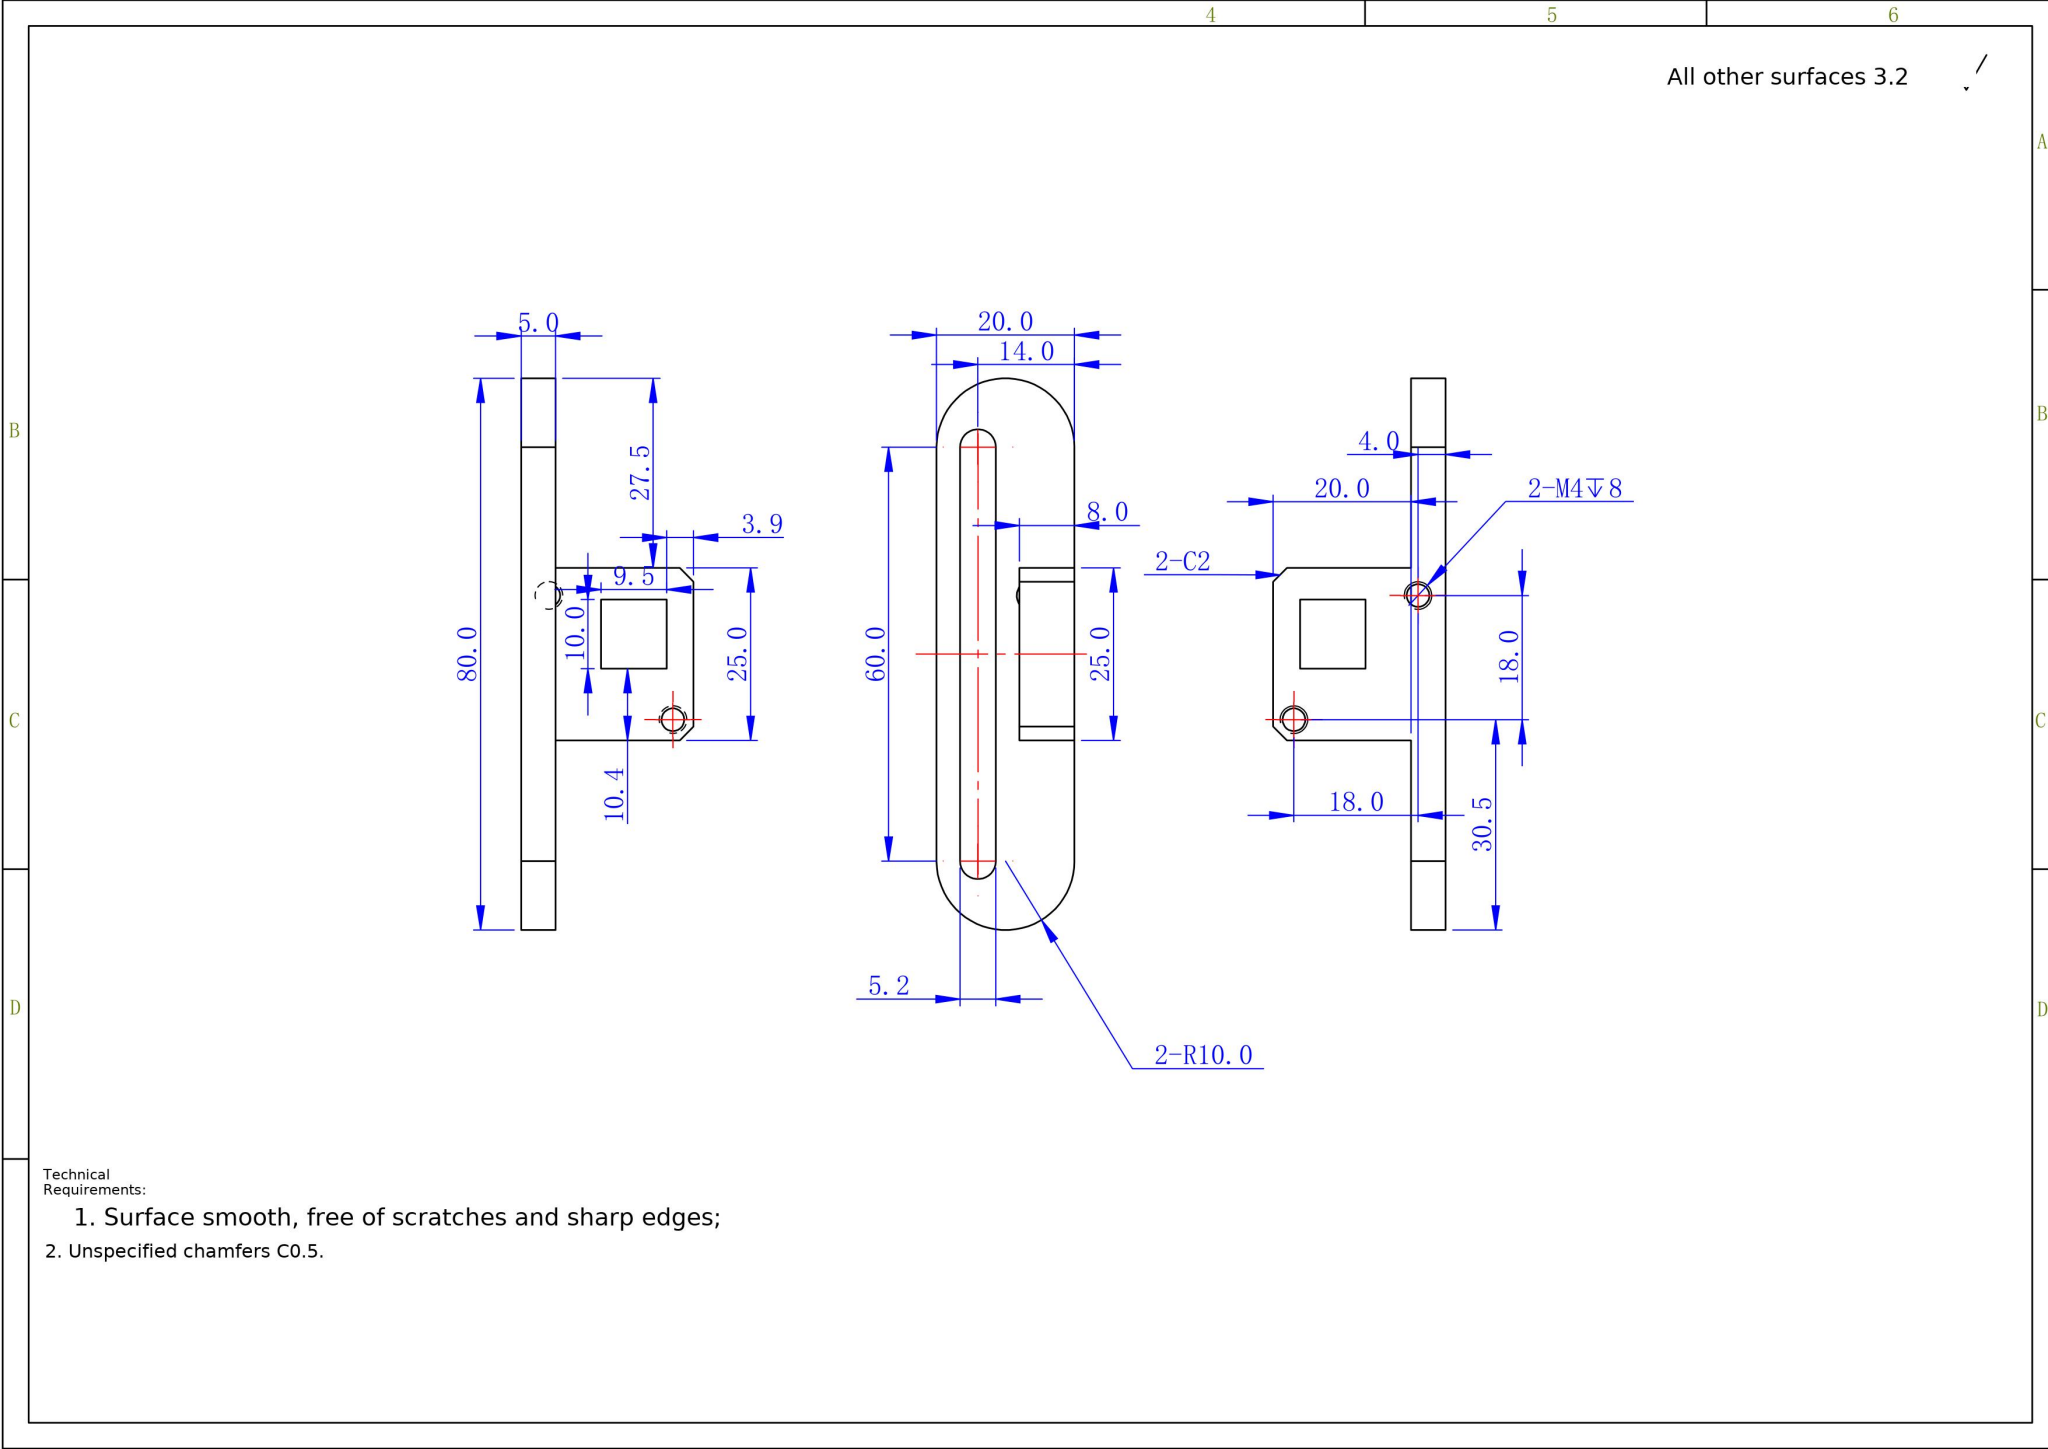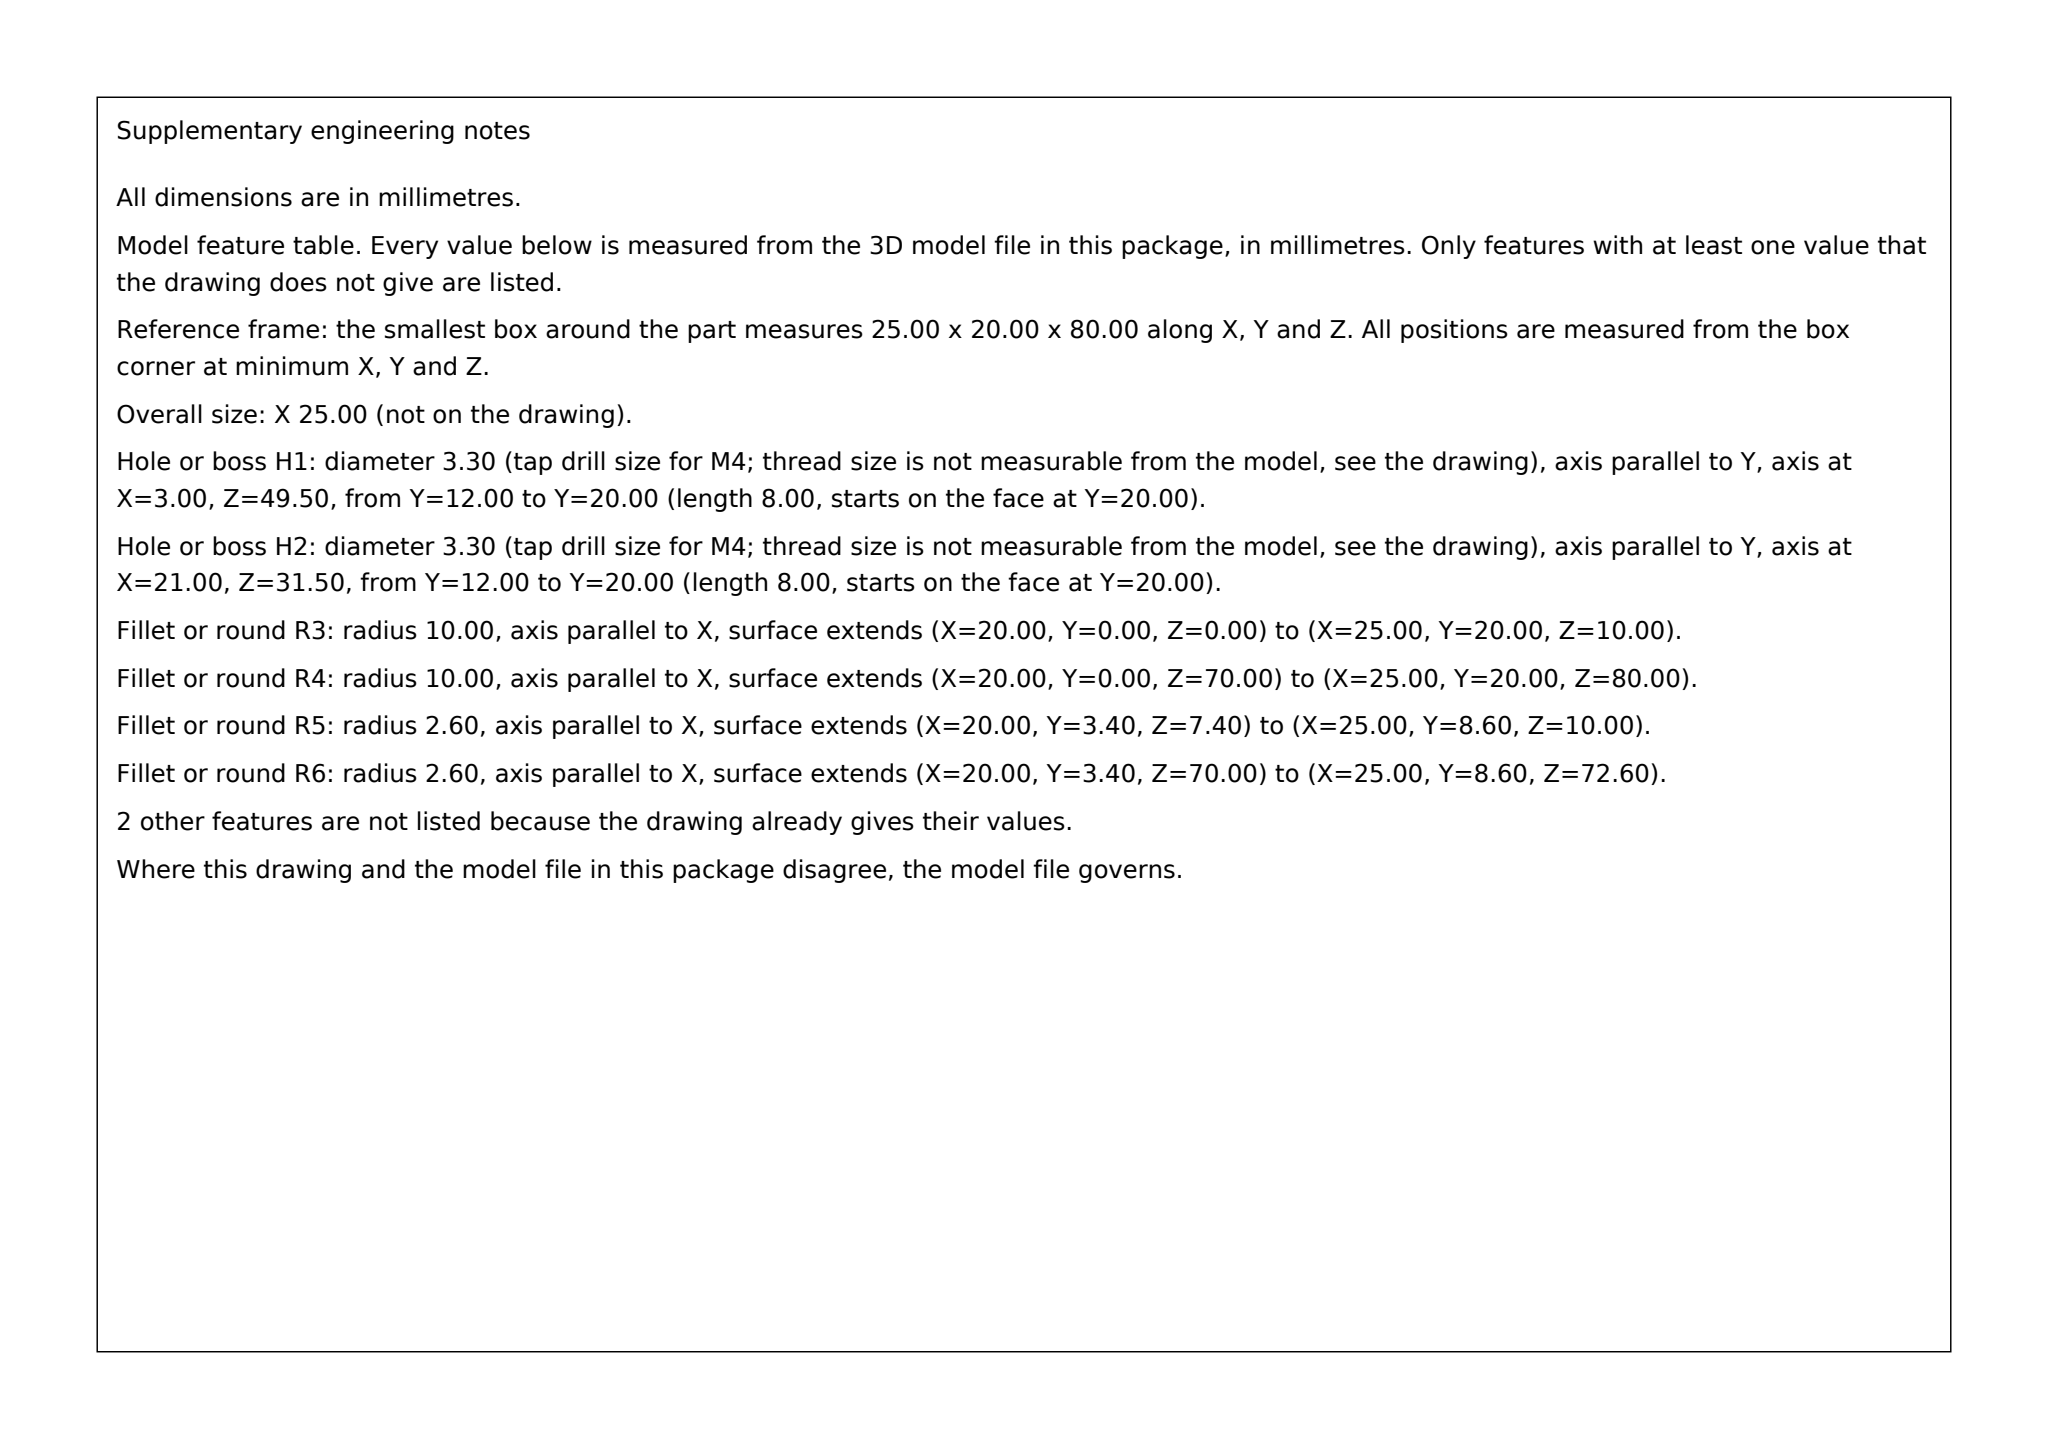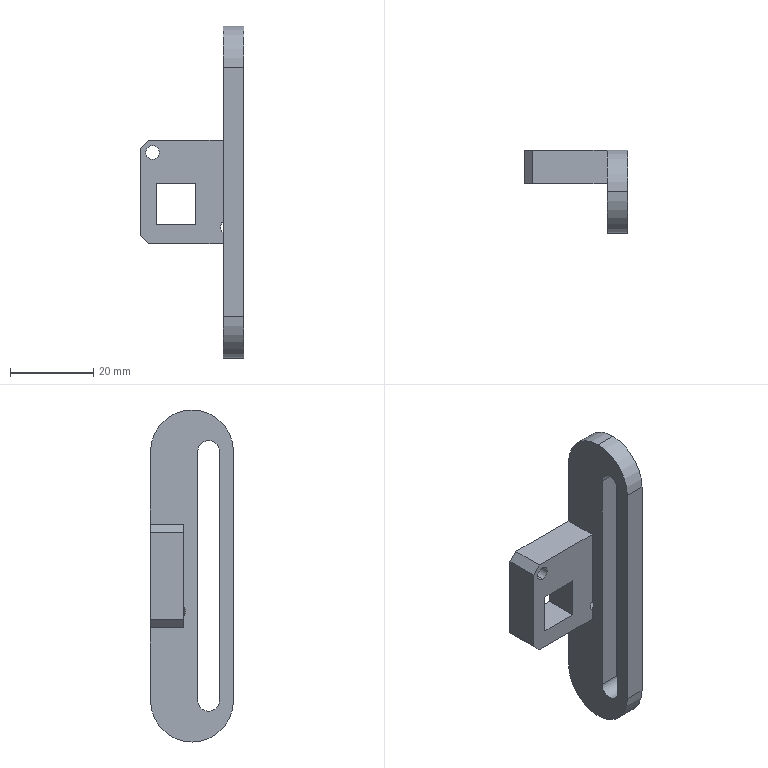Part | SolidWorks | mm | 1 solid | 29 faces | box 25 x 20 x 80 mm | volume 8973 mm3 | plane 16 | cylinder 11 | cone 2 | commonest cylinder face diameters 3.3 x4 20 x4 5.2 x3